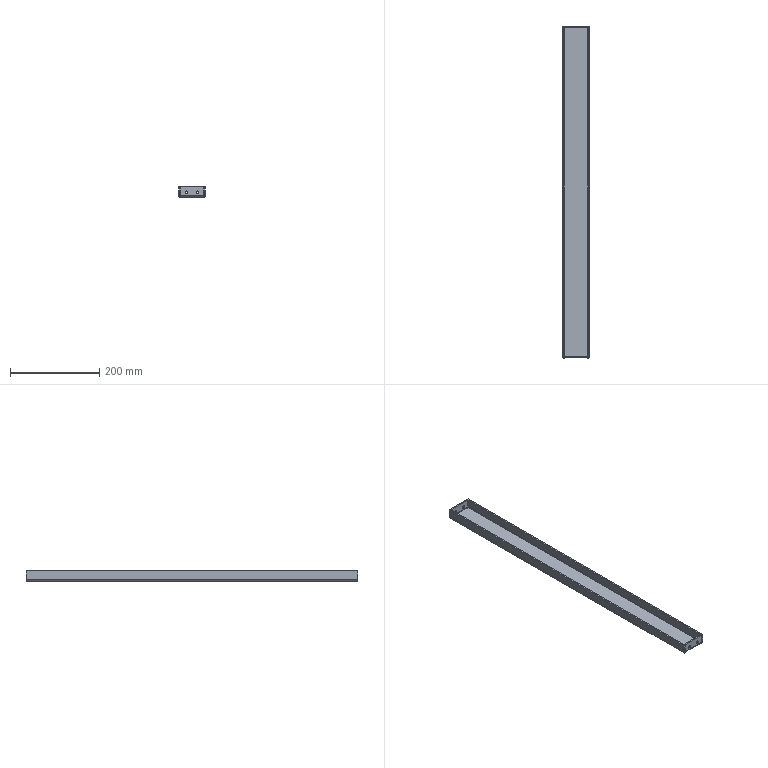Component | SolidWorks | Beam(No.30)-1 | 1 solid | 58 faces | volume 224496 mm3 | plane 42 | cylinder 16 | commonest cylinder face diameters 6.5 x8 8 x4 2 x4 | material Plain Carbon Steel